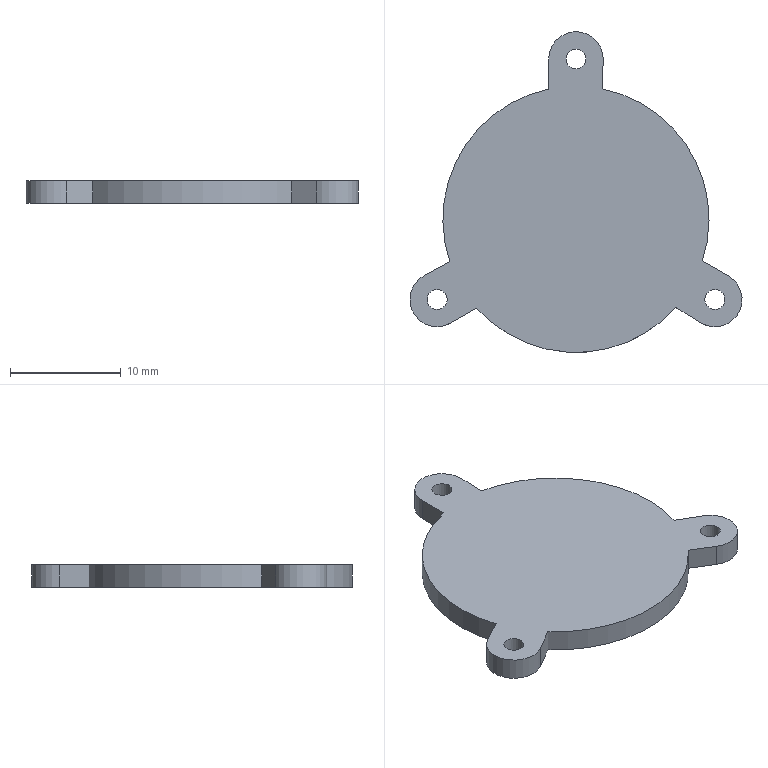Component | NX | ATOMIZER_MOUNT | 1 solid | 17 faces | volume 1021 mm3 | cylinder 9 | plane 8 | commonest cylinder face diameters 4.915 x3 24 x3 1.8 x3